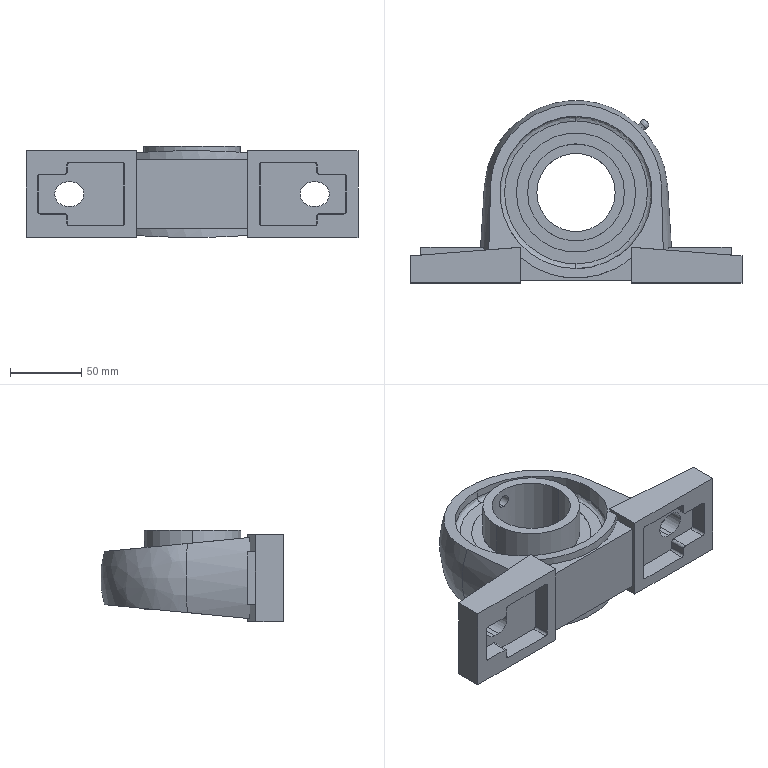Component | SolidWorks | BearingHousing-1 | 1 solid | 121 faces | volume 500870 mm3 | plane 58 | cylinder 28 | spline 19 | cone 16 | commonest cylinder face diameters 106.905 x6 83.84 x6 68.05 x6 17 x4 8.918 x2 55 x2 120.242 x2